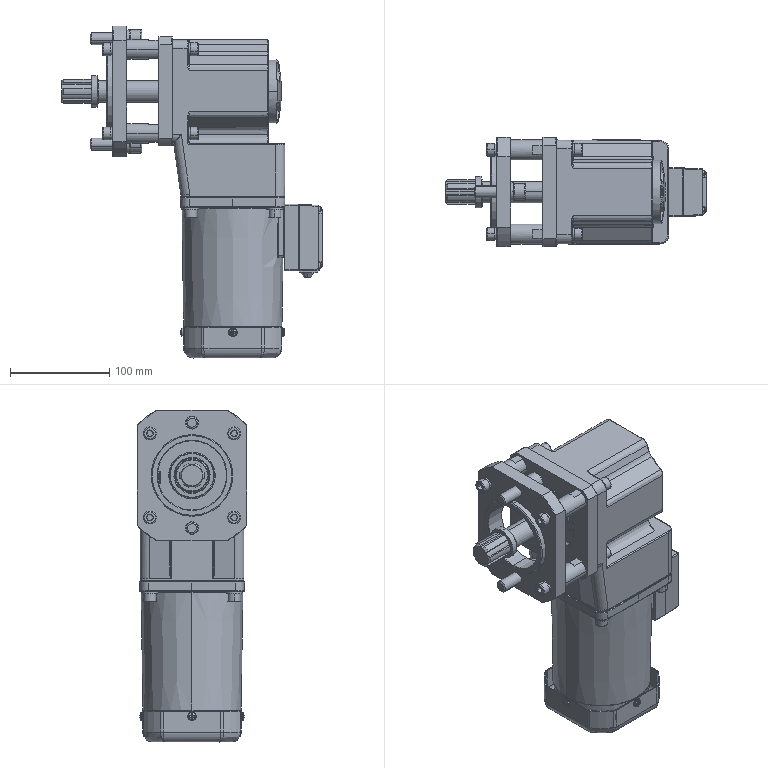Assembly | SolidWorks | mm | 32 component files | 35 solids | 3231 faces | box 263.1 x 110 x 335 mm | volume 2279457 mm3 | cylinder 991 | spline 877 | plane 849 | cone 456 | torus 58 | commonest cylinder face diameters 0.5 x131 2 x110 8 x60 1 x54 3 x54 4 x52 9 x32 13 x30
Bill of materials:
100YS200GV22+100GF10RC F707 | 1 |  | Multi-body housing assembly: a blocky upper housing with a bolted flange face and a round cover with radial ribs, a stepped middle block, a long roughly cylindrical/faceted body below it, a rounded end cap, and a small rectangular box with a cover mounted on the side of the body.
12_T93 | 2 | Plain Carbon Steel | Split ring washer with a rectangular cross-section and a single radial gap.
8_T93 | 8 | Plain Carbon Steel | Split ring washer with a rectangular cross-section and a single radial gap; looks the same as unnamed part.
M12_40_T70.1 | 2 | Plain Carbon Steel | Cap-head screw shape: a cylindrical head with a hexagonal socket and rounded top edge, and a plain cylindrical shank with a chamfered tip.
M8_25_T70.1 | 4 | Plain Carbon Steel | Cap-head screw shape with a cylindrical head and a shorter plain cylindrical shank with a chamfered tip; the renders show mostly the underside of the head and the shank end.
M8_45_T70.1 | 4 | Plain Carbon Steel | Long, slender cap-head screw shape: a cylindrical head with a hexagonal socket and a long plain shank with a chamfered tip.
XXXXX08-01-040511 | 1 | Q235-A | Flat flange plate with chamfered corners, a large central bore, and a raised circular pilot boss on one side; it has four counterbored corner holes and two plain holes on the vertical centerline.
XXXXX08-01-040512 | 1 | Q235-A | Flat square plate with chamfered corners, a large central circular hole, and four corner through-holes.
XXXXX08-01-040513 | 4 | 45 | Cylindrical sleeve with a central through-bore and chamfered ends; one end has a reduced section with a flat on one side.
22_T894.1 | 2 | 65Mn | Thin open ring with two lugs at the gap, each with a small hole; looks like an external retaining ring.
6_28 A_T1096 | 1 |  | Rectangular bar with fully rounded ends and slightly rounded edges; looks like a round-ended parallel key.
XXXXX08-01-040514 | 1 | 45 | Cylindrical shaft with a toothed (splined or gear-like) section at one end and two shallow circumferential grooves or lines along the plain body; both ends are chamfered.
XXXXX08-01-040515 | 1 | 45 | Plain flat annular ring (washer/spacer-like shape): a short hollow cylinder with flat parallel faces, a concentric circular through-bore, and smooth cylindrical outer and inner walls.
Mates:
1. coincident | XXXXX08-01-040511-1 face at (-14, 75, 0) dir (-1, 0, 0) | 8_T93-1 face at (-14, 42.426, 42.426) dir (1, 0, 0)
2. concentric | XXXXX08-01-040511-1 face at (-14, 42.426, 42.426) dir (-1, 0, 0) r 4.5 | 8_T93-1 face at (-16.1, 42.426, 42.426) dir (1, 0, 0) r 4.05
3. coincident | 8_T93-1 face at (-16.1, 42.426, 42.426) dir (-1, 0, 0) | M8_25_T70.1-1 face at (-16.1, 48.926, 42.426) dir (1, 0, 0)
4. concentric | 8_T93-1 face at (-16.1, 42.426, 42.426) dir (1, 0, 0) r 4.05 | M8_25_T70.1-1 face at (-24.1, 42.426, 42.426) dir (-1, 0, 0) r 4
5. coincident | XXXXX08-01-040511-1 face at (0, 35, 0) dir (1, 0, 0) | 12_T93-1 face at (0, 0, -53.2) dir (-1, 0, 0)
6. concentric | XXXXX08-01-040511-1 face at (0, 0, -53.2) dir (1, 0, 0) r 6.5 | 12_T93-1 face at (0, 0, -53.2) dir (1, 0, 0) r 6.1
7. coincident | 12_T93-1 face at (3.1, 0, -53.2) dir (1, 0, 0) | M12_40_T70.1-1 face at (3.1, 3.437, -61.518) dir (-1, 0, 0)
8. concentric | 12_T93-1 face at (0, 0, -53.2) dir (1, 0, 0) r 6.1 | M12_40_T70.1-1 face at (15.1, 0, -53.2) dir (1, 0, 0) r 6
9. concentric | XXXXX08-01-040511-1 face at (-4, -42.426, -42.426) dir (1, 0, 0) r 10 | XXXXX08-01-040512-1 face at (36, -42.426, -42.426) dir (-1, 0, 0) r 10
10. concentric | XXXXX08-01-040511-1 face at (-4, 42.426, 42.426) dir (1, 0, 0) r 10 | XXXXX08-01-040512-1 face at (36, 42.426, 42.426) dir (-1, 0, 0) r 10
11. concentric | XXXXX08-01-040511-1 face at (-4, 42.426, 42.426) dir (1, 0, 0) r 10 | XXXXX08-01-040513-1 face at (-4, 42.426, 42.426) dir (1, 0, 0) r 10
12. coincident | XXXXX08-01-040511-1 face at (-4, 42.426, 42.426) dir (1, 0, 0) | XXXXX08-01-040513-1 face at (-4, 42.426, 42.426) dir (-1, 0, 0)
13. parallel | XXXXX08-01-040512-1 face at (32, -47.236, 55) dir (0, 0, 1) | XXXXX08-01-040513-1 face at (36, 52.426, 51.426) dir (0, 0, 1)
14. coincident | XXXXX08-01-040512-1 face at (36, 42.426, 42.426) dir (-1, 0, 0) | XXXXX08-01-040513-1 face at (36, 42.426, 42.426) dir (1, 0, 0)
15. coincident | 8_T93-5 face at (64.1, 42.426, 42.426) dir (1, 0, 0) | M8_45_T70.1-1 face at (64.1, 44.908, 36.419) dir (-1, 0, 0)
16. concentric | 8_T93-5 face at (62, 42.426, 42.426) dir (1, 0, 0) r 4.05 | M8_45_T70.1-1 face at (72.1, 42.426, 42.426) dir (1, 0, 0) r 4
17. concentric | XXXXX08-01-040514RotaryDriveShaft-1/XXXXX08-01-040514-1 face at (77.3, 0, 0) dir (1, 0, 0) r 11 | 100YS200GV22+100GF10RC F707-1 face at (77.5, 0, 0) dir (-1, 0, 0) r 11
18. concentric | XXXXX08-01-040512-1 face at (46, 42.426, 42.426) dir (1, 0, 0) r 4.5 | 100YS200GV22+100GF10RC F707-1 face at (61.436, 42.426, 42.426) dir (-1, 0, 0) r 4.5
19. coincident | XXXXX08-01-040512-1 face at (46, 0, 0) dir (1, 0, 0) | 100YS200GV22+100GF10RC F707-1 face at (46, -54.495, -54.496) dir (-1, 0, 0)
20. concentric | M8_45_T70.1-1 face at (72.1, 42.426, 42.426) dir (1, 0, 0) r 4 | 100YS200GV22+100GF10RC F707-1 face at (61.436, 42.426, 42.426) dir (-1, 0, 0) r 4.5
21. coincident | 8_T93-5 face at (62, 42.426, 42.426) dir (-1, 0, 0) | 100YS200GV22+100GF10RC F707-1 face at (62, 53.4, -53.517) dir (1, 0, 0)
22. concentric | XXXXX08-01-040514-1 face at (143, 0, 0) dir (1, 0, 0) r 11 | XXXXX08-01-040515-1 face at (36, 0, 0) dir (-1, 0, 0) r 11.1
23. coincident | XXXXX08-01-040514-1 face at (30, 12.65, 0) dir (1, 0, 0) | XXXXX08-01-040515-1 face at (30, 0, 0) dir (-1, 0, 0)
24. coincident | XXXXX08-01-040514-1 face at (114, 7.5, 0) dir (0, 1, 0) | 6_28 A_T1096-1 face at (114, 7.5, 0) dir (0, -1, 0)
25. concentric | XXXXX08-01-040514-1 face at (136, 12.65, 0) dir (0, -1, 0) r 3 | 6_28 A_T1096-1 face at (136, 7.5, 0) dir (0, 1, 0) r 3
26. concentric | XXXXX08-01-040514-1 face at (114, 12.65, 0) dir (0, -1, 0) r 3 | 6_28 A_T1096-1 face at (114, 7.5, 0) dir (0, 1, 0) r 3
27. concentric | XXXXX08-01-040514-1 face at (143, 0, 0) dir (1, 0, 0) r 11 | 22_T894.1-1 face at (37, 0, 0) dir (-1, 0, 0) r 10.5
28. coincident | XXXXX08-01-040514-1 face at (36, 11, 0) dir (1, 0, 0) | 22_T894.1-1 face at (36, -9.221, 8.817) dir (-1, 0, 0)
29. concentric | XXXXX08-01-040514-1 face at (143, 0, 0) dir (1, 0, 0) r 10.5 | 22_T894.1-2 face at (107.9, 0, 0) dir (-1, 0, 0) r 10.5
30. coincident | XXXXX08-01-040514-1 face at (106.9, 11, 0) dir (1, 0, 0) | 22_T894.1-2 face at (106.9, -9.221, 8.817) dir (-1, 0, 0)